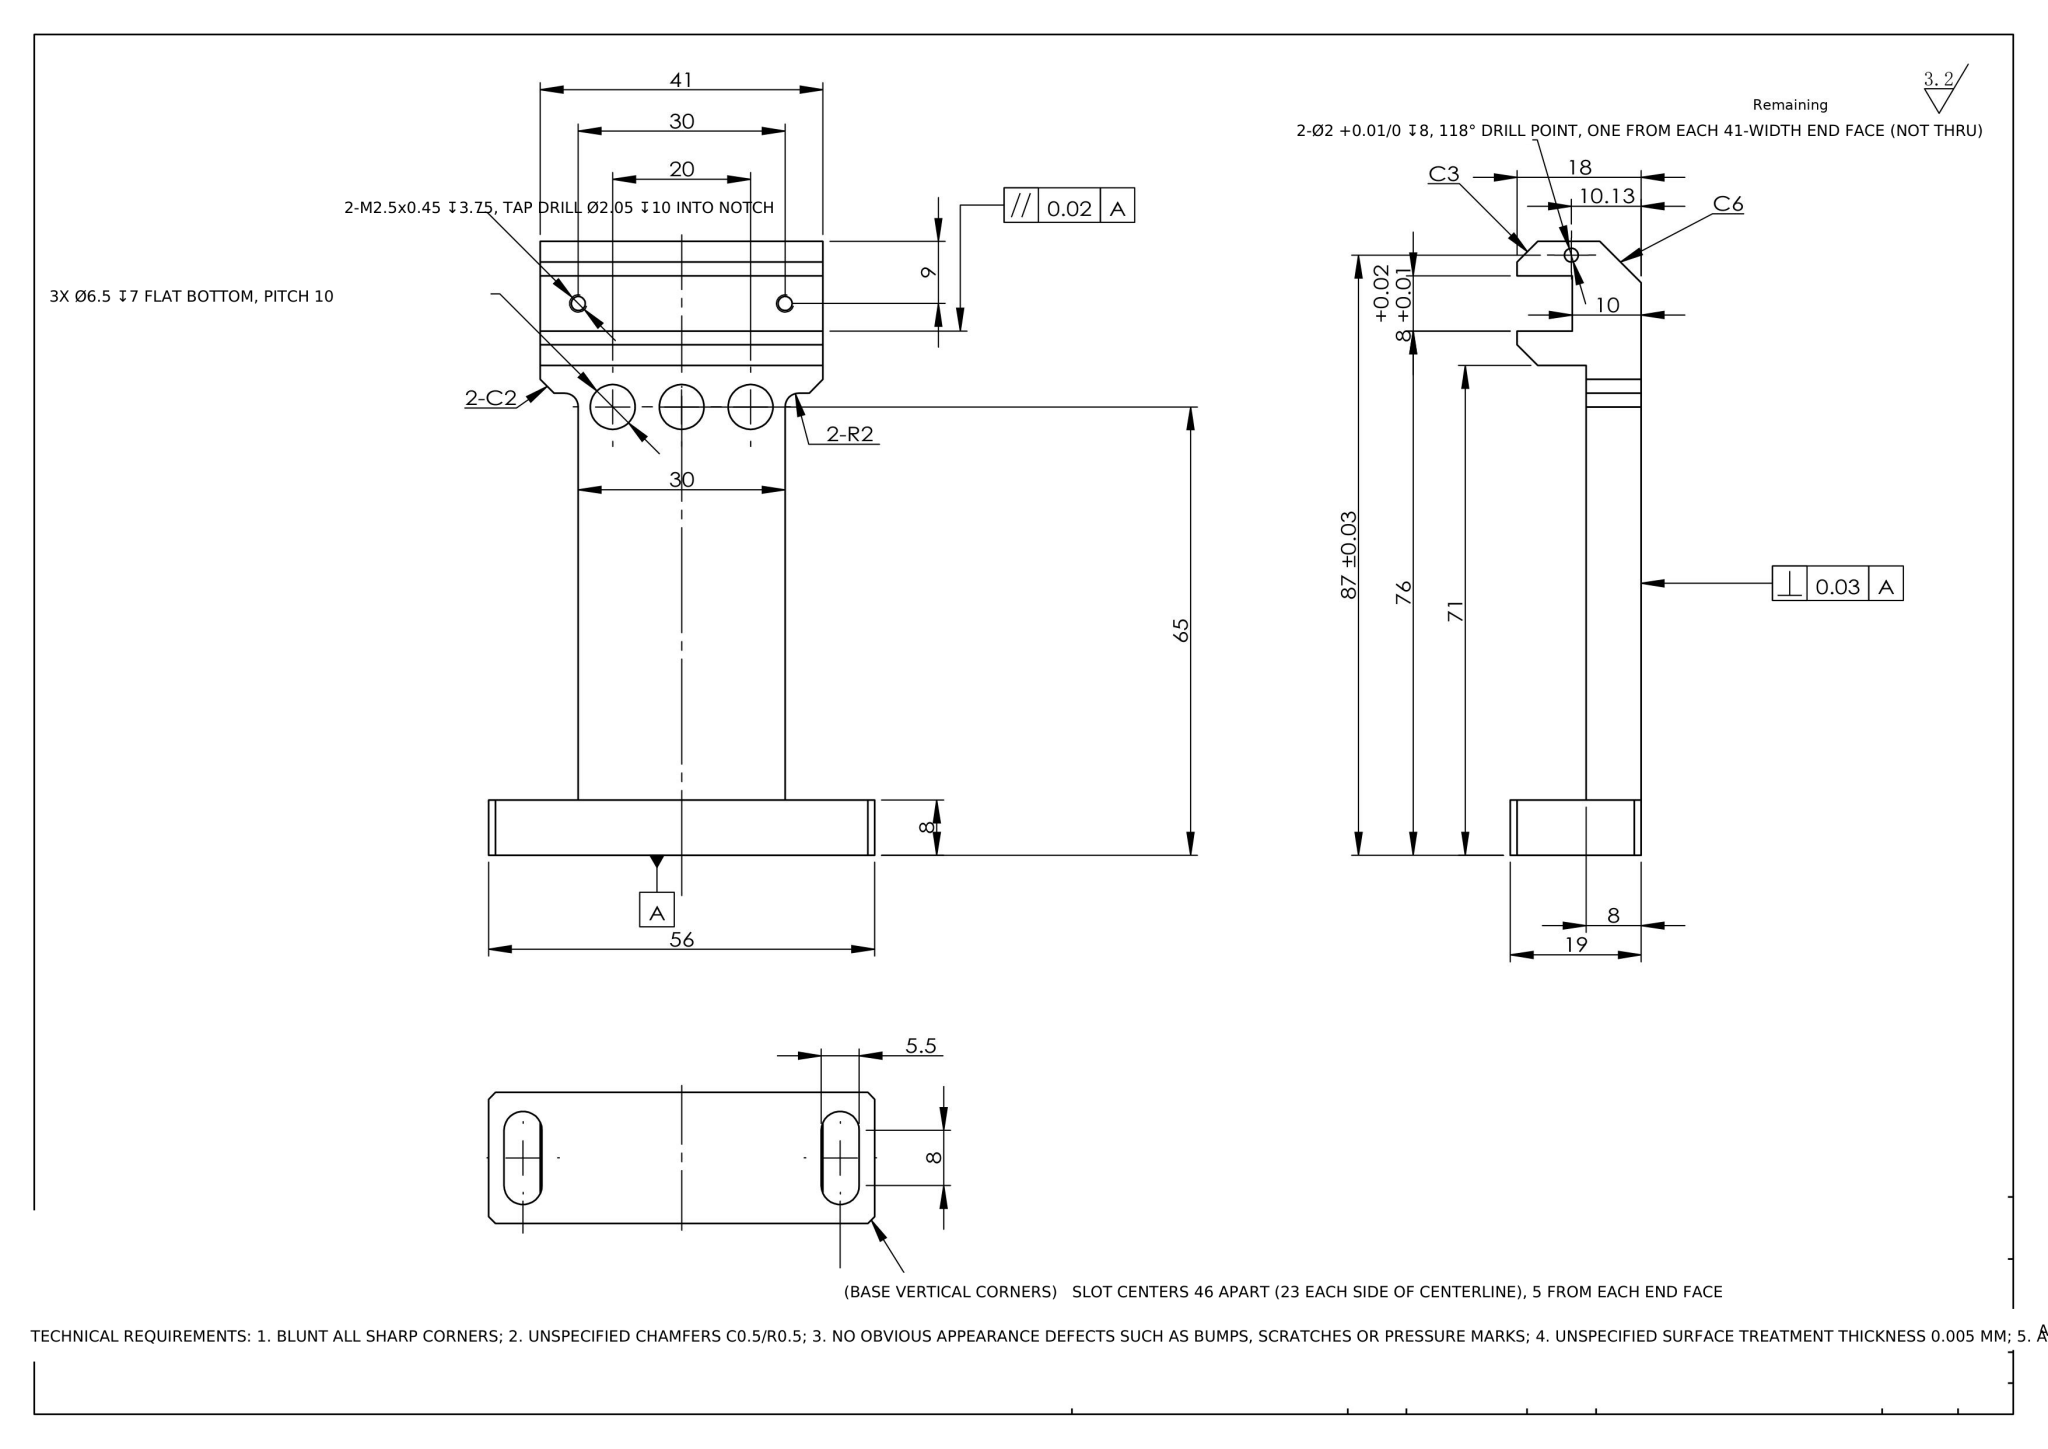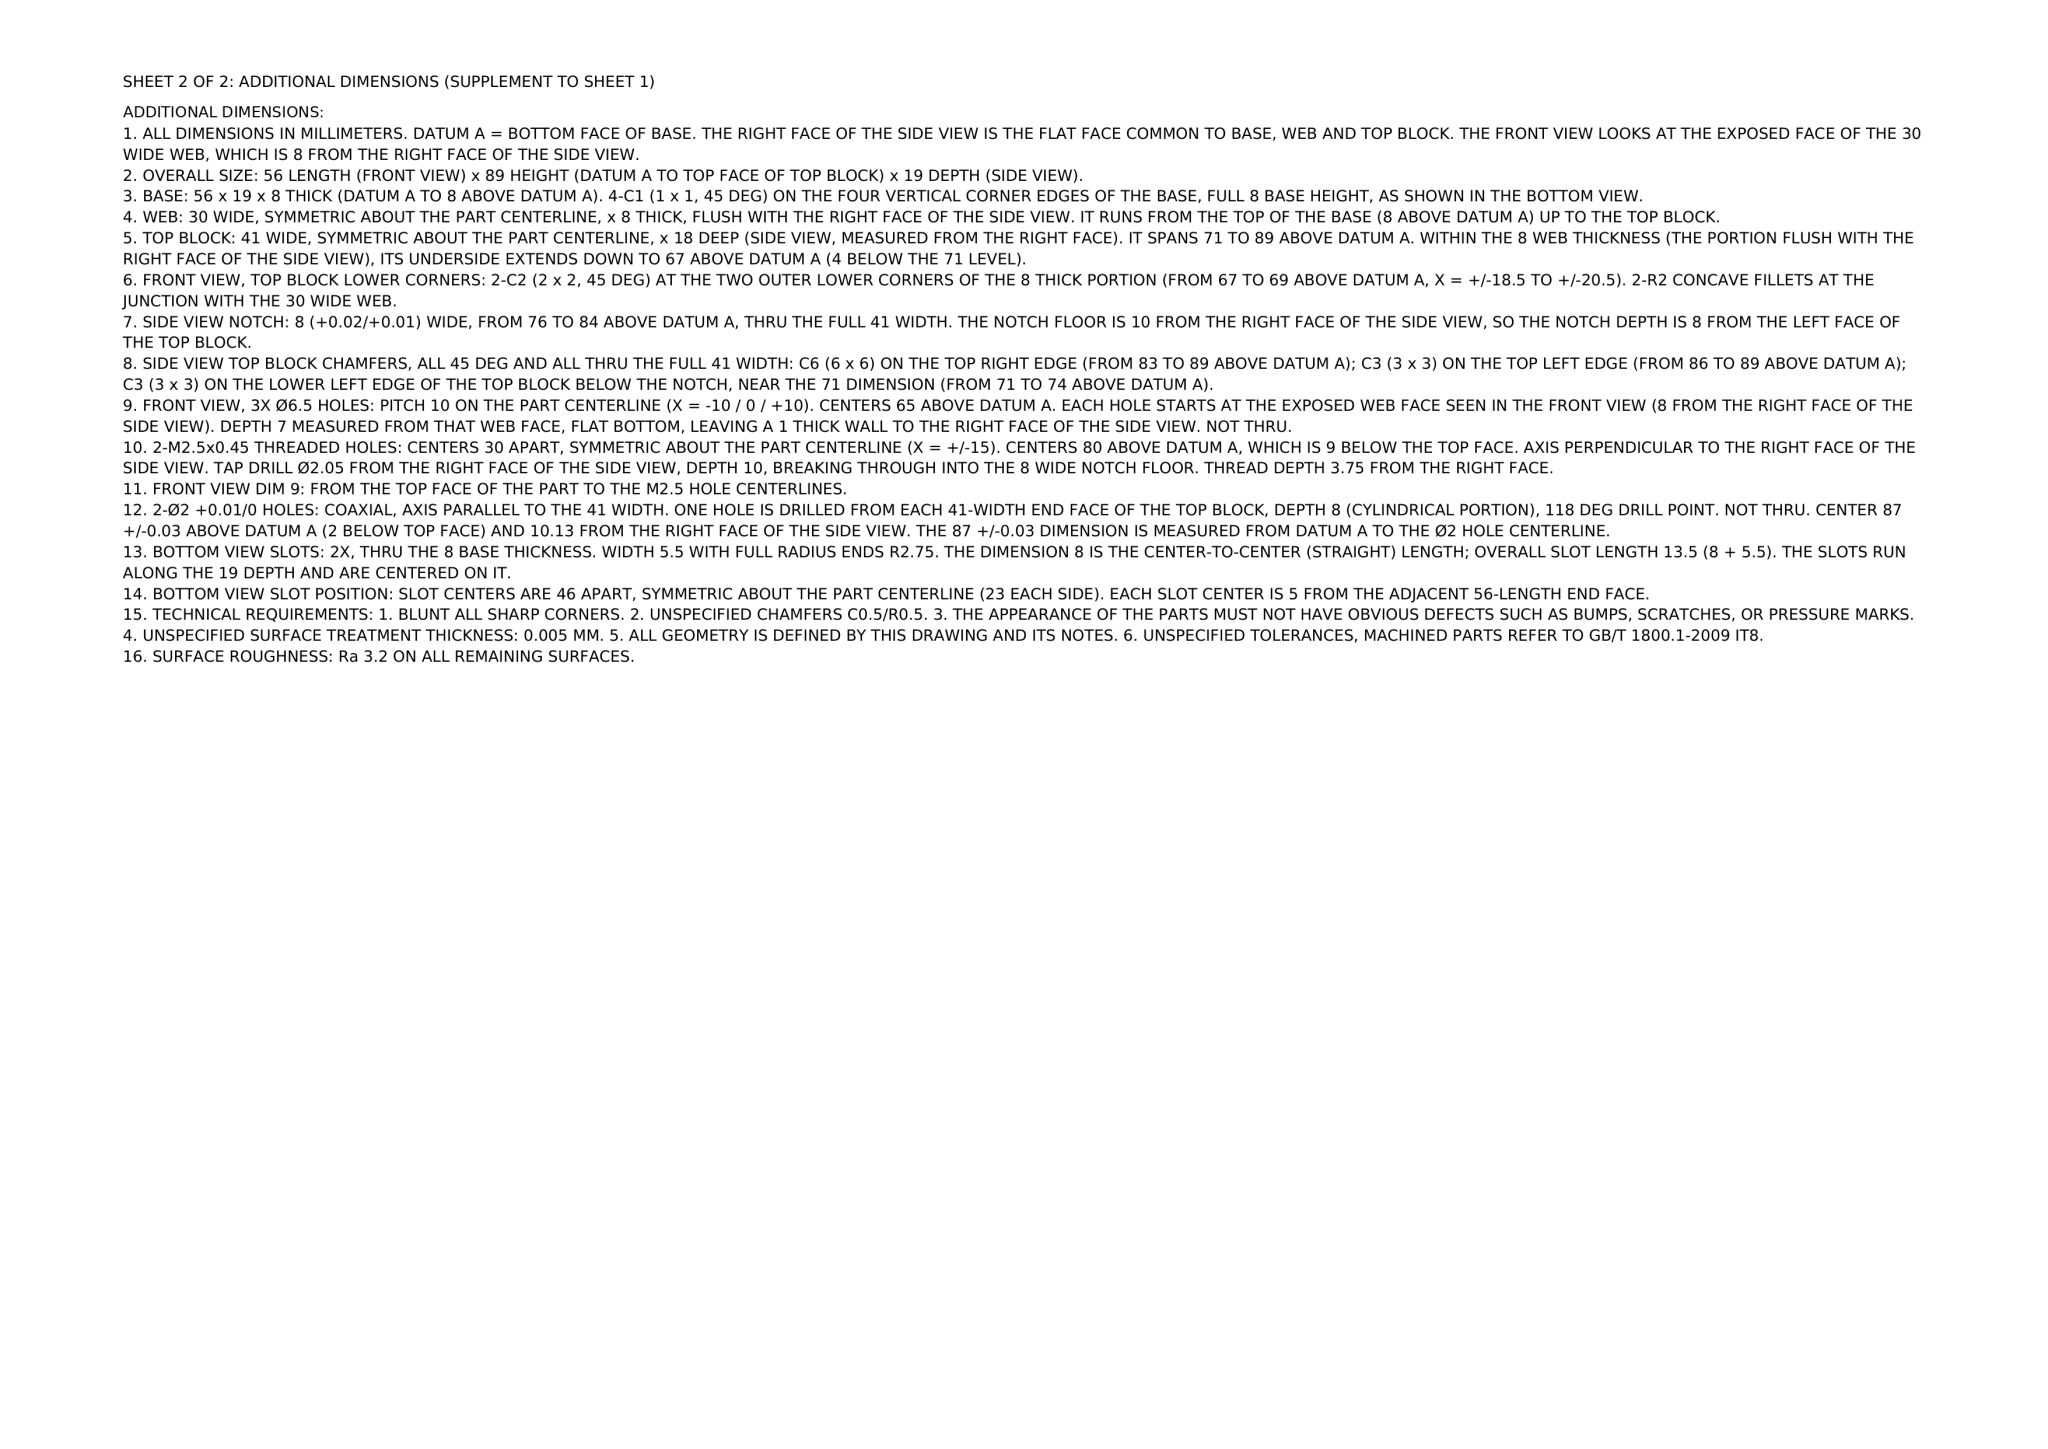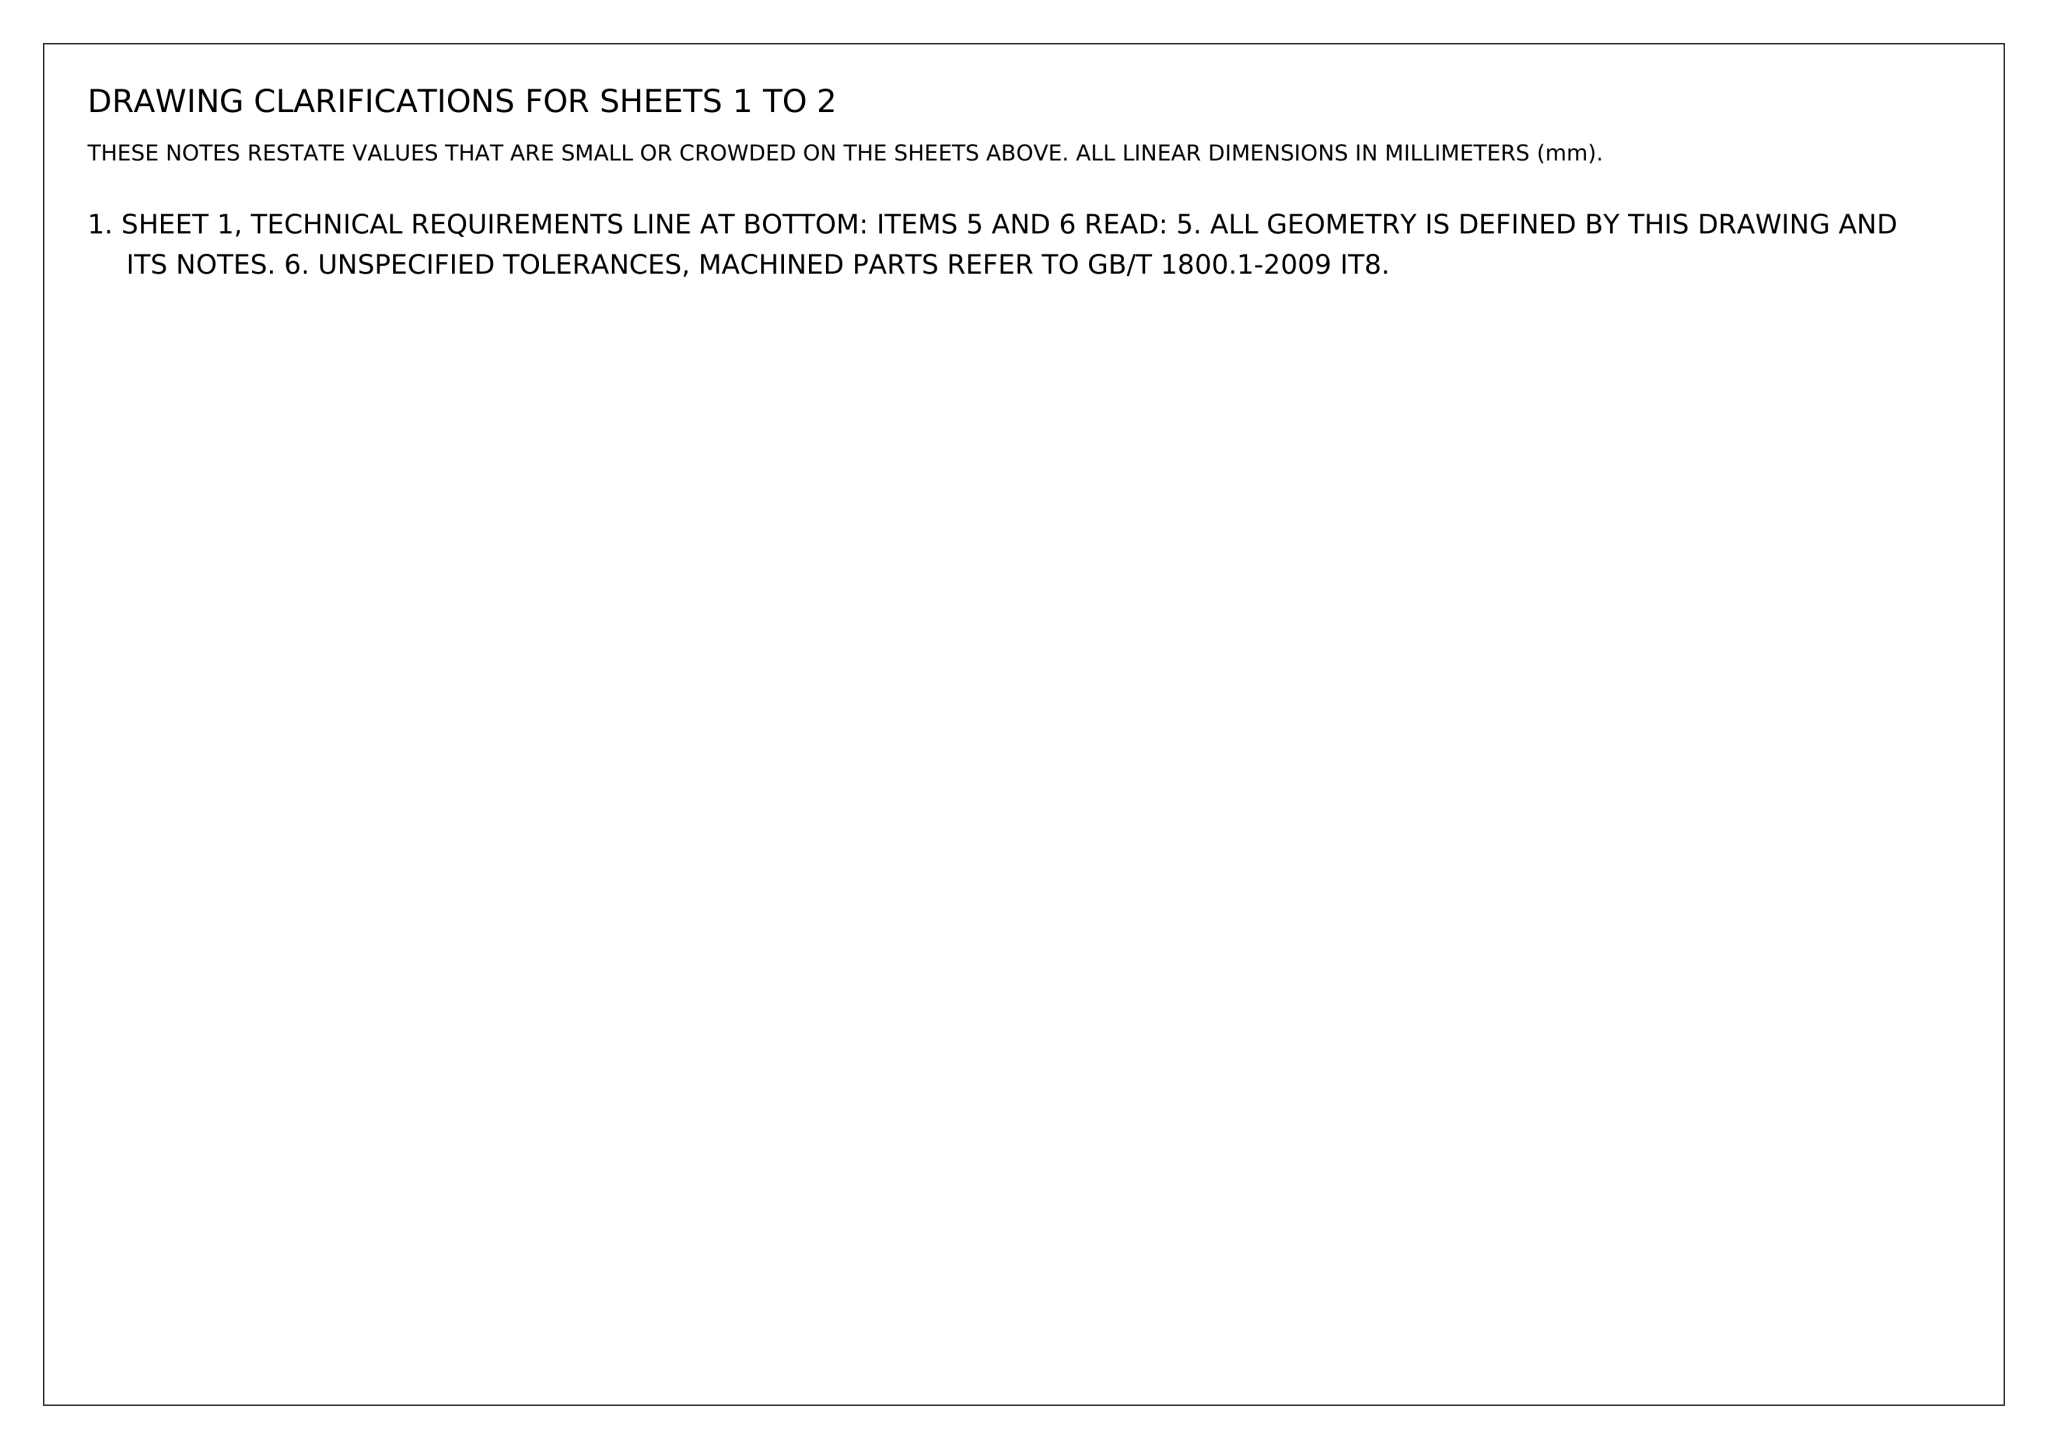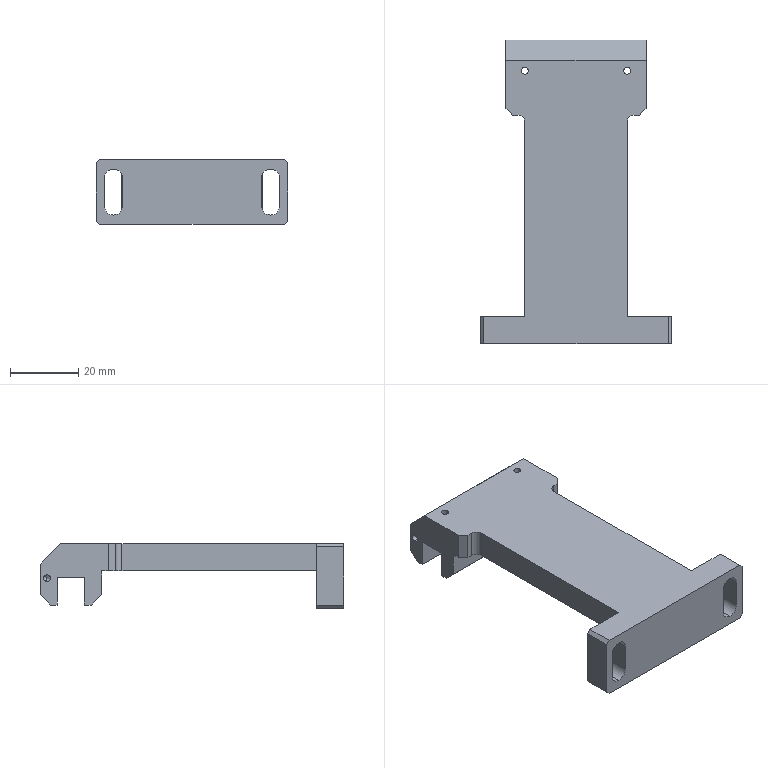Part | NX | mm | 1 solid | 62 faces | box 56 x 89 x 19 mm | volume 31604 mm3 | plane 36 | cylinder 22 | cone 4 | commonest cylinder face diameters 5.5 x6 6.5 x6 2.05 x4 2 x4 4 x2